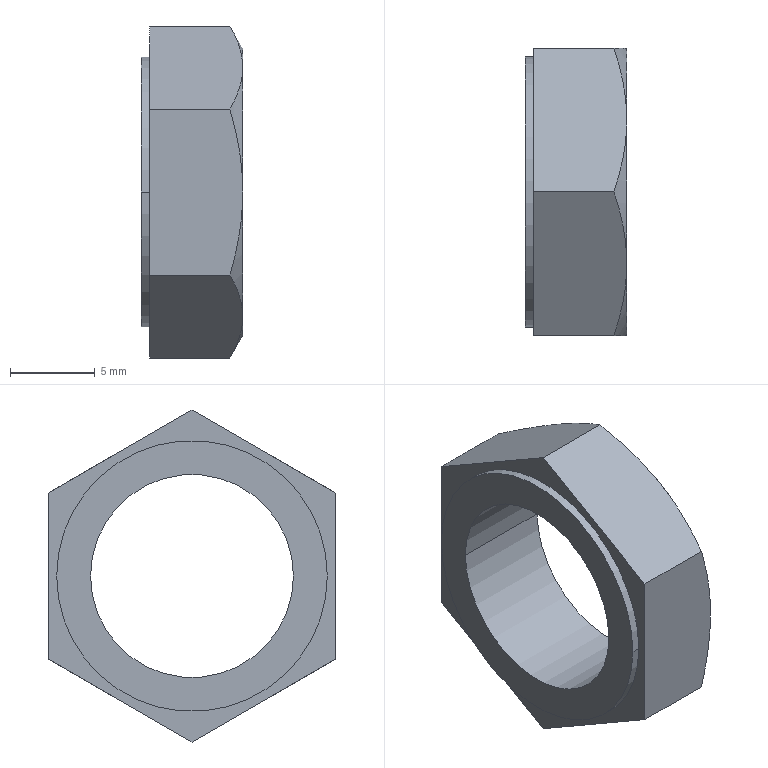Component | SolidWorks | MI10x10U(0)+()-1_MI10-M12x1_25 - Nut-1 | 1 solid | 19 faces | box 6 x 17 x 19.63 mm | volume 793 mm3 | plane 9 | cone 6 | cylinder 4 | commonest cylinder face diameters 12 x2 16 x2
build123d program:
from build123d import *

# Parameters (mm, degrees)
SKETCH2_W                         = 34
SKETCH2_H                         = 34
CUT_EXTRUDE1_DEPTH                = 12
SKETCH1_R                         = 6
M12_THREAD_MAJOR_DIA_RELIEF_DEPTH = 15.303


with BuildPart() as part:
    # Sketch1_2 → Revolve1 (revolve)
    with BuildSketch(Plane.XY, mode=Mode.PRIVATE) as revolve1_sk:
        Polygon((0, 0), (0, 8.5), (0.9815, 10.2), (5.5, 10.2), (5.5, 8), (6, 8), (6, 0), align=None)
    revolve(revolve1_sk.sketch.rotate(Axis((6, 0, 0), (-1, 0, 0)), 270), axis=Axis((6, 0, 0), (-1, 0, 0)))

    # Sketch2 → Cut-Extrude1 (cut)
    with BuildSketch(Plane(origin=(0, 0, 0), x_dir=(0, 0, -1), z_dir=(1, 0, 0))):
        Rectangle(SKETCH2_W, SKETCH2_H)
        Polygon((-8.5, -4.907), (0, -9.815), (8.5, -4.907), (8.5, 4.907), (0, 9.815), (-8.5, 4.907), align=None, mode=Mode.SUBTRACT)
    extrude(amount=CUT_EXTRUDE1_DEPTH, mode=Mode.SUBTRACT)

    # Sketch3 → Cut-Revolve1 (revolve, cut)
    with BuildSketch(Plane.XY, mode=Mode.PRIVATE) as cut_revolve1_sk:
        Polygon((0, 0), (0, 6), (0.6765, 5.324), (5.324, 5.324), (6, 6), (6, 0), align=None)
    revolve(cut_revolve1_sk.sketch.rotate(Axis((6, 0, 0), (-1, 0, 0)), 270), axis=Axis((6, 0, 0), (-1, 0, 0)), mode=Mode.SUBTRACT)

    # Sketch1 → M12 thread major-dia relief (cut, through all)
    with BuildSketch(Plane.ZY):
        Circle(SKETCH1_R)
    extrude(amount=-M12_THREAD_MAJOR_DIA_RELIEF_DEPTH, mode=Mode.SUBTRACT)


solid = part.part

# Placed as in the assembly
solid = solid.moved(Location((-7.325, 30.452, 72.77), (-90, 0, 180)))
STEP:
#1=CARTESIAN_POINT('',(-0.5246,0.9627,2.865));
#2=VERTEX_POINT('',#1);
#3=CARTESIAN_POINT('',(-0.5246,1.435,2.865));
#4=VERTEX_POINT('',#3);
#5=CARTESIAN_POINT('',(-0.5246,1.199,2.865));
#6=DIRECTION('',(1.,-0.,-0.));
#7=DIRECTION('',(0.,1.,0.));
#8=AXIS2_PLACEMENT_3D('',#5,#6,#7);
#9=CIRCLE('',#8,0.2362);
#10=EDGE_CURVE('',#2,#4,#9,.T.);
#11=ORIENTED_EDGE('',*,*,#10,.F.);
#12=CARTESIAN_POINT('',(-0.2884,0.9627,2.865));
#13=VERTEX_POINT('',#12);
#14=CARTESIAN_POINT('',(-0.5246,0.9627,2.865));
#15=DIRECTION('',(1.,-0.,-0.));
#16=VECTOR('',#15,39.37);
#17=LINE('',#14,#16);
#18=EDGE_CURVE('',#2,#13,#17,.T.);
#19=ORIENTED_EDGE('',*,*,#18,.T.);
#20=CARTESIAN_POINT('',(-0.2884,1.435,2.865));
#21=VERTEX_POINT('',#20);
#22=CARTESIAN_POINT('',(-0.2884,1.199,2.865));
#23=DIRECTION('',(1.,-0.,-0.));
#24=DIRECTION('',(0.,1.,0.));
#25=AXIS2_PLACEMENT_3D('',#22,#23,#24);
#26=CIRCLE('',#25,0.2362);
#27=EDGE_CURVE('',#13,#21,#26,.T.);
#28=ORIENTED_EDGE('',*,*,#27,.T.);
#29=CARTESIAN_POINT('',(-0.5246,1.435,2.865));
#30=DIRECTION('',(1.,-0.,-0.));
#31=VECTOR('',#30,39.37);
#32=LINE('',#29,#31);
#33=EDGE_CURVE('',#4,#21,#32,.T.);
#34=ORIENTED_EDGE('',*,*,#33,.F.);
#35=EDGE_LOOP('',(#11,#19,#28,#34));
#36=FACE_OUTER_BOUND('',#35,.T.);
#37=CARTESIAN_POINT('',(-0.5246,1.199,2.865));
#38=DIRECTION('',(1.,-0.,-0.));
#39=DIRECTION('',(0.,1.,0.));
#40=AXIS2_PLACEMENT_3D('',#37,#38,#39);
#41=CYLINDRICAL_SURFACE('',#40,0.2362);
#42=ADVANCED_FACE('',(#36),#41,.F.);
#43=CARTESIAN_POINT('',(-0.5246,1.514,2.865));
#44=VERTEX_POINT('',#43);
#45=CARTESIAN_POINT('',(-0.5246,0.8839,2.865));
#46=VERTEX_POINT('',#45);
#47=CARTESIAN_POINT('',(-0.5246,1.199,2.865));
#48=DIRECTION('',(1.,-0.,-0.));
#49=DIRECTION('',(0.,1.,0.));
#50=AXIS2_PLACEMENT_3D('',#47,#48,#49);
#51=CIRCLE('',#50,0.315);
#52=EDGE_CURVE('',#44,#46,#51,.T.);
#53=ORIENTED_EDGE('',*,*,#52,.T.);
#54=CARTESIAN_POINT('',(-0.5049,0.8839,2.865));
#55=VERTEX_POINT('',#54);
#56=CARTESIAN_POINT('',(-0.5246,0.8839,2.865));
#57=DIRECTION('',(1.,-0.,-0.));
#58=VECTOR('',#57,39.37);
#59=LINE('',#56,#58);
#60=EDGE_CURVE('',#46,#55,#59,.T.);
#61=ORIENTED_EDGE('',*,*,#60,.T.);
#62=CARTESIAN_POINT('',(-0.5049,1.514,2.865));
#63=VERTEX_POINT('',#62);
#64=CARTESIAN_POINT('',(-0.5049,1.199,2.865));
#65=DIRECTION('',(1.,-0.,-0.));
#66=DIRECTION('',(0.,1.,0.));
#67=AXIS2_PLACEMENT_3D('',#64,#65,#66);
#68=CIRCLE('',#67,0.315);
#69=EDGE_CURVE('',#63,#55,#68,.T.);
#70=ORIENTED_EDGE('',*,*,#69,.F.);
#71=CARTESIAN_POINT('',(-0.5246,1.514,2.865));
#72=DIRECTION('',(1.,-0.,-0.));
#73=VECTOR('',#72,39.37);
#74=LINE('',#71,#73);
#75=EDGE_CURVE('',#44,#63,#74,.T.);
#76=ORIENTED_EDGE('',*,*,#75,.F.);
#77=EDGE_LOOP('',(#53,#61,#70,#76));
#78=FACE_OUTER_BOUND('',#77,.T.);
#79=CARTESIAN_POINT('',(-0.5246,1.199,2.865));
#80=DIRECTION('',(1.,-0.,-0.));
#81=DIRECTION('',(0.,1.,0.));
#82=AXIS2_PLACEMENT_3D('',#79,#80,#81);
#83=CYLINDRICAL_SURFACE('',#82,0.315);
#84=ADVANCED_FACE('',(#78),#83,.T.);
#85=CARTESIAN_POINT('',(-0.5049,1.199,3.251));
#86=VERTEX_POINT('',#85);
#87=CARTESIAN_POINT('',(-0.5049,1.534,3.058));
#88=VERTEX_POINT('',#87);
#89=CARTESIAN_POINT('',(-0.5049,1.192,3.255));
#90=DIRECTION('',(0.,0.866,-0.5));
#91=VECTOR('',#90,39.37);
#92=LINE('',#89,#91);
#93=EDGE_CURVE('',#86,#88,#92,.T.);
#94=ORIENTED_EDGE('',*,*,#93,.T.);
#95=CARTESIAN_POINT('',(-0.5049,1.534,2.672));
#96=VERTEX_POINT('',#95);
#97=CARTESIAN_POINT('',(-0.5049,1.534,3.267));
#98=DIRECTION('',(-0.,0.,-1.));
#99=VECTOR('',#98,39.37);
#100=LINE('',#97,#99);
#101=EDGE_CURVE('',#88,#96,#100,.T.);
#102=ORIENTED_EDGE('',*,*,#101,.T.);
#103=CARTESIAN_POINT('',(-0.5049,1.199,2.479));
#104=VERTEX_POINT('',#103);
#105=CARTESIAN_POINT('',(-0.5049,1.54,2.676));
#106=DIRECTION('',(-0.,-0.866,-0.5));
#107=VECTOR('',#106,39.37);
#108=LINE('',#105,#107);
#109=EDGE_CURVE('',#96,#104,#108,.T.);
#110=ORIENTED_EDGE('',*,*,#109,.T.);
#111=CARTESIAN_POINT('',(-0.5049,0.8643,2.672));
#112=VERTEX_POINT('',#111);
#113=CARTESIAN_POINT('',(-0.5049,0.8577,2.676));
#114=DIRECTION('',(-0.,-0.866,0.5));
#115=VECTOR('',#114,39.37);
#116=LINE('',#113,#115);
#117=EDGE_CURVE('',#104,#112,#116,.T.);
#118=ORIENTED_EDGE('',*,*,#117,.T.);
#119=CARTESIAN_POINT('',(-0.5049,0.8643,3.058));
#120=VERTEX_POINT('',#119);
#121=CARTESIAN_POINT('',(-0.5049,0.8643,3.267));
#122=DIRECTION('',(0.,-0.,1.));
#123=VECTOR('',#122,39.37);
#124=LINE('',#121,#123);
#125=EDGE_CURVE('',#112,#120,#124,.T.);
#126=ORIENTED_EDGE('',*,*,#125,.T.);
#127=CARTESIAN_POINT('',(-0.5049,1.205,3.255));
#128=DIRECTION('',(0.,0.866,0.5));
#129=VECTOR('',#128,39.37);
#130=LINE('',#127,#129);
#131=EDGE_CURVE('',#120,#86,#130,.T.);
#132=ORIENTED_EDGE('',*,*,#131,.T.);
#133=EDGE_LOOP('',(#94,#102,#110,#118,#126,#132));
#134=FACE_OUTER_BOUND('',#133,.T.);
#135=ORIENTED_EDGE('',*,*,#69,.T.);
#136=CARTESIAN_POINT('',(-0.5049,1.199,2.865));
#137=DIRECTION('',(1.,-0.,-0.));
#138=DIRECTION('',(0.,1.,0.));
#139=AXIS2_PLACEMENT_3D('',#136,#137,#138);
#140=CIRCLE('',#139,0.315);
#141=EDGE_CURVE('',#55,#63,#140,.T.);
#142=ORIENTED_EDGE('',*,*,#141,.T.);
#143=EDGE_LOOP('',(#135,#142));
#144=FACE_BOUND('',#143,.T.);
#145=CARTESIAN_POINT('',(-0.5049,1.199,3.267));
#146=DIRECTION('',(1.,-0.,-0.));
#147=DIRECTION('',(0.,1.,0.));
#148=AXIS2_PLACEMENT_3D('',#145,#146,#147);
#149=PLANE('',#148);
#150=ADVANCED_FACE('',(#134,#144),#149,.F.);
#151=ORIENTED_EDGE('',*,*,#60,.F.);
#152=CARTESIAN_POINT('',(-0.5246,1.199,2.865));
#153=DIRECTION('',(1.,-0.,-0.));
#154=DIRECTION('',(0.,1.,0.));
#155=AXIS2_PLACEMENT_3D('',#152,#153,#154);
#156=CIRCLE('',#155,0.315);
#157=EDGE_CURVE('',#46,#44,#156,.T.);
#158=ORIENTED_EDGE('',*,*,#157,.T.);
#159=ORIENTED_EDGE('',*,*,#75,.T.);
#160=ORIENTED_EDGE('',*,*,#141,.F.);
#161=EDGE_LOOP('',(#151,#158,#159,#160));
#162=FACE_OUTER_BOUND('',#161,.T.);
#163=CARTESIAN_POINT('',(-0.5246,1.199,2.865));
#164=DIRECTION('',(1.,-0.,-0.));
#165=DIRECTION('',(0.,1.,0.));
#166=AXIS2_PLACEMENT_3D('',#163,#164,#165);
#167=CYLINDRICAL_SURFACE('',#166,0.315);
#168=ADVANCED_FACE('',(#162),#167,.T.);
#169=CARTESIAN_POINT('',(-0.5246,1.199,2.865));
#170=DIRECTION('',(1.,-0.,-0.));
#171=DIRECTION('',(0.,1.,0.));
#172=AXIS2_PLACEMENT_3D('',#169,#170,#171);
#173=CIRCLE('',#172,0.2362);
#174=EDGE_CURVE('',#4,#2,#173,.T.);
#175=ORIENTED_EDGE('',*,*,#174,.T.);
#176=ORIENTED_EDGE('',*,*,#10,.T.);
#177=EDGE_LOOP('',(#175,#176));
#178=FACE_BOUND('',#177,.T.);
#179=ORIENTED_EDGE('',*,*,#52,.F.);
#180=ORIENTED_EDGE('',*,*,#157,.F.);
#181=EDGE_LOOP('',(#179,#180));
#182=FACE_OUTER_BOUND('',#181,.T.);
#183=CARTESIAN_POINT('',(-0.5246,1.199,3.18));
#184=DIRECTION('',(1.,-0.,-0.));
#185=DIRECTION('',(0.,1.,0.));
#186=AXIS2_PLACEMENT_3D('',#183,#184,#185);
#187=PLANE('',#186);
#188=ADVANCED_FACE('',(#178,#182),#187,.F.);
#189=CARTESIAN_POINT('',(-0.3183,1.534,2.672));
#190=VERTEX_POINT('',#189);
#191=CARTESIAN_POINT('',(-0.7608,1.534,2.672));
#192=DIRECTION('',(1.,-0.,-0.));
#193=VECTOR('',#192,39.37);
#194=LINE('',#191,#193);
#195=EDGE_CURVE('',#96,#190,#194,.T.);
#196=ORIENTED_EDGE('',*,*,#195,.F.);
#197=ORIENTED_EDGE('',*,*,#101,.F.);
#198=CARTESIAN_POINT('',(-0.3183,1.534,3.058));
#199=VERTEX_POINT('',#198);
#200=CARTESIAN_POINT('',(-0.7608,1.534,3.058));
#201=DIRECTION('',(1.,-0.,-0.));
#202=VECTOR('',#201,39.37);
#203=LINE('',#200,#202);
#204=EDGE_CURVE('',#88,#199,#203,.T.);
#205=ORIENTED_EDGE('',*,*,#204,.T.);
#206=CARTESIAN_POINT('',(-0.2884,1.534,2.865));
#207=VERTEX_POINT('',#206);
#208=CARTESIAN_POINT('',(-0.2884,1.534,2.865));
#209=CARTESIAN_POINT('',(-0.2884,1.534,2.898));
#210=CARTESIAN_POINT('',(-0.2913,1.534,2.931));
#211=CARTESIAN_POINT('',(-0.3018,1.534,2.995));
#212=CARTESIAN_POINT('',(-0.3093,1.534,3.027));
#213=CARTESIAN_POINT('',(-0.3183,1.534,3.058));
#214=B_SPLINE_CURVE_WITH_KNOTS('',3,(#208,#209,#210,#211,#212,#213),.UNSPECIFIED.,.F.,.F.,(4,2,4),(0.01375,0.01624,0.01872),.UNSPECIFIED.);
#215=EDGE_CURVE('',#207,#199,#214,.T.);
#216=ORIENTED_EDGE('',*,*,#215,.F.);
#217=CARTESIAN_POINT('',(-0.3183,1.534,2.672));
#218=CARTESIAN_POINT('',(-0.3092,1.534,2.703));
#219=CARTESIAN_POINT('',(-0.3016,1.534,2.735));
#220=CARTESIAN_POINT('',(-0.2912,1.534,2.8));
#221=CARTESIAN_POINT('',(-0.2884,1.534,2.832));
#222=CARTESIAN_POINT('',(-0.2884,1.534,2.865));
#223=B_SPLINE_CURVE_WITH_KNOTS('',3,(#217,#218,#219,#220,#221,#222),.UNSPECIFIED.,.F.,.F.,(4,2,4),(0.00879,0.01127,0.01375),.UNSPECIFIED.);
#224=EDGE_CURVE('',#190,#207,#223,.T.);
#225=ORIENTED_EDGE('',*,*,#224,.F.);
#226=EDGE_LOOP('',(#196,#197,#205,#216,#225));
#227=FACE_OUTER_BOUND('',#226,.T.);
#228=CARTESIAN_POINT('',(-0.7608,1.534,3.058));
#229=DIRECTION('',(-0.,-1.,-0.));
#230=DIRECTION('',(1.,-0.,-0.));
#231=AXIS2_PLACEMENT_3D('',#228,#229,#230);
#232=PLANE('',#231);
#233=ADVANCED_FACE('',(#227),#232,.F.);
#234=CARTESIAN_POINT('',(-0.3183,1.199,2.479));
#235=VERTEX_POINT('',#234);
#236=CARTESIAN_POINT('',(-0.7608,1.199,2.479));
#237=DIRECTION('',(1.,-0.,-0.));
#238=VECTOR('',#237,39.37);
#239=LINE('',#236,#238);
#240=EDGE_CURVE('',#104,#235,#239,.T.);
#241=ORIENTED_EDGE('',*,*,#240,.F.);
#242=ORIENTED_EDGE('',*,*,#109,.F.);
#243=ORIENTED_EDGE('',*,*,#195,.T.);
#244=CARTESIAN_POINT('',(-0.2884,1.366,2.575));
#245=VERTEX_POINT('',#244);
#246=CARTESIAN_POINT('',(-0.2884,1.366,2.575));
#247=CARTESIAN_POINT('',(-0.2884,1.38,2.583));
#248=CARTESIAN_POINT('',(-0.2891,1.395,2.592));
#249=CARTESIAN_POINT('',(-0.2918,1.423,2.608));
#250=CARTESIAN_POINT('',(-0.2939,1.437,2.616));
#251=CARTESIAN_POINT('',(-0.3017,1.479,2.64));
#252=CARTESIAN_POINT('',(-0.3092,1.506,2.656));
#253=CARTESIAN_POINT('',(-0.3183,1.534,2.672));
#254=B_SPLINE_CURVE_WITH_KNOTS('',3,(#246,#247,#248,#249,#250,#251,#252,#253),.UNSPECIFIED.,.F.,.F.,(4,2,2,4),(0.004966,0.006203,0.007439,0.009913),.UNSPECIFIED.);
#255=EDGE_CURVE('',#245,#190,#254,.T.);
#256=ORIENTED_EDGE('',*,*,#255,.F.);
#257=CARTESIAN_POINT('',(-0.3183,1.199,2.479));
#258=CARTESIAN_POINT('',(-0.3092,1.226,2.494));
#259=CARTESIAN_POINT('',(-0.3017,1.254,2.51));
#260=CARTESIAN_POINT('',(-0.2913,1.31,2.542));
#261=CARTESIAN_POINT('',(-0.2884,1.338,2.559));
#262=CARTESIAN_POINT('',(-0.2884,1.366,2.575));
#263=B_SPLINE_CURVE_WITH_KNOTS('',3,(#257,#258,#259,#260,#261,#262),.UNSPECIFIED.,.F.,.F.,(4,2,4),(0.00000024,0.002483,0.004966),.UNSPECIFIED.);
#264=EDGE_CURVE('',#235,#245,#263,.T.);
#265=ORIENTED_EDGE('',*,*,#264,.F.);
#266=EDGE_LOOP('',(#241,#242,#243,#256,#265));
#267=FACE_OUTER_BOUND('',#266,.T.);
#268=CARTESIAN_POINT('',(-0.7608,1.534,2.672));
#269=DIRECTION('',(0.,-0.5,0.866));
#270=DIRECTION('',(0.,0.866,0.5));
#271=AXIS2_PLACEMENT_3D('',#268,#269,#270);
#272=PLANE('',#271);
#273=ADVANCED_FACE('',(#267),#272,.F.);
#274=CARTESIAN_POINT('',(-0.3183,0.8643,2.672));
#275=VERTEX_POINT('',#274);
#276=CARTESIAN_POINT('',(-0.7608,0.8643,2.672));
#277=DIRECTION('',(1.,-0.,-0.));
#278=VECTOR('',#277,39.37);
#279=LINE('',#276,#278);
#280=EDGE_CURVE('',#112,#275,#279,.T.);
#281=ORIENTED_EDGE('',*,*,#280,.F.);
#282=ORIENTED_EDGE('',*,*,#117,.F.);
#283=ORIENTED_EDGE('',*,*,#240,.T.);
#284=CARTESIAN_POINT('',(-0.2884,1.032,2.575));
#285=VERTEX_POINT('',#284);
#286=CARTESIAN_POINT('',(-0.2884,1.032,2.575));
#287=CARTESIAN_POINT('',(-0.2884,1.046,2.567));
#288=CARTESIAN_POINT('',(-0.2891,1.06,2.559));
#289=CARTESIAN_POINT('',(-0.2918,1.088,2.542));
#290=CARTESIAN_POINT('',(-0.2939,1.102,2.534));
#291=CARTESIAN_POINT('',(-0.3017,1.144,2.51));
#292=CARTESIAN_POINT('',(-0.3092,1.172,2.494));
#293=CARTESIAN_POINT('',(-0.3183,1.199,2.479));
#294=B_SPLINE_CURVE_WITH_KNOTS('',3,(#286,#287,#288,#289,#290,#291,#292,#293),.UNSPECIFIED.,.F.,.F.,(4,2,2,4),(0.004966,0.006203,0.007439,0.009913),.UNSPECIFIED.);
#295=EDGE_CURVE('',#285,#235,#294,.T.);
#296=ORIENTED_EDGE('',*,*,#295,.F.);
#297=CARTESIAN_POINT('',(-0.3183,0.8643,2.672));
#298=CARTESIAN_POINT('',(-0.3092,0.8916,2.656));
#299=CARTESIAN_POINT('',(-0.3017,0.9192,2.64));
#300=CARTESIAN_POINT('',(-0.2913,0.9749,2.608));
#301=CARTESIAN_POINT('',(-0.2884,1.003,2.592));
#302=CARTESIAN_POINT('',(-0.2884,1.032,2.575));
#303=B_SPLINE_CURVE_WITH_KNOTS('',3,(#297,#298,#299,#300,#301,#302),.UNSPECIFIED.,.F.,.F.,(4,2,4),(0.00000024,0.002483,0.004966),.UNSPECIFIED.);
#304=EDGE_CURVE('',#275,#285,#303,.T.);
#305=ORIENTED_EDGE('',*,*,#304,.F.);
#306=EDGE_LOOP('',(#281,#282,#283,#296,#305));
#307=FACE_OUTER_BOUND('',#306,.T.);
#308=CARTESIAN_POINT('',(-0.7608,1.199,2.479));
#309=DIRECTION('',(0.,0.5,0.866));
#310=DIRECTION('',(0.,0.866,-0.5));
#311=AXIS2_PLACEMENT_3D('',#308,#309,#310);
#312=PLANE('',#311);
#313=ADVANCED_FACE('',(#307),#312,.F.);
#314=CARTESIAN_POINT('',(-0.3183,0.8643,3.058));
#315=VERTEX_POINT('',#314);
#316=CARTESIAN_POINT('',(-0.7608,0.8643,3.058));
#317=DIRECTION('',(1.,-0.,-0.));
#318=VECTOR('',#317,39.37);
#319=LINE('',#316,#318);
#320=EDGE_CURVE('',#120,#315,#319,.T.);
#321=ORIENTED_EDGE('',*,*,#320,.F.);
#322=ORIENTED_EDGE('',*,*,#125,.F.);
#323=ORIENTED_EDGE('',*,*,#280,.T.);
#324=CARTESIAN_POINT('',(-0.2884,0.8643,2.865));
#325=VERTEX_POINT('',#324);
#326=CARTESIAN_POINT('',(-0.2884,0.8643,2.865));
#327=CARTESIAN_POINT('',(-0.2884,0.8643,2.832));
#328=CARTESIAN_POINT('',(-0.2912,0.8643,2.8));
#329=CARTESIAN_POINT('',(-0.3016,0.8643,2.735));
#330=CARTESIAN_POINT('',(-0.3092,0.8643,2.703));
#331=CARTESIAN_POINT('',(-0.3183,0.8643,2.672));
#332=B_SPLINE_CURVE_WITH_KNOTS('',3,(#326,#327,#328,#329,#330,#331),.UNSPECIFIED.,.F.,.F.,(4,2,4),(0.02652,0.029,0.03149),.UNSPECIFIED.);
#333=EDGE_CURVE('',#325,#275,#332,.T.);
#334=ORIENTED_EDGE('',*,*,#333,.F.);
#335=CARTESIAN_POINT('',(-0.3183,0.8643,3.058));
#336=CARTESIAN_POINT('',(-0.3093,0.8643,3.027));
#337=CARTESIAN_POINT('',(-0.3018,0.8643,2.995));
#338=CARTESIAN_POINT('',(-0.2913,0.8643,2.931));
#339=CARTESIAN_POINT('',(-0.2884,0.8643,2.898));
#340=CARTESIAN_POINT('',(-0.2884,0.8643,2.865));
#341=B_SPLINE_CURVE_WITH_KNOTS('',3,(#335,#336,#337,#338,#339,#340),.UNSPECIFIED.,.F.,.F.,(4,2,4),(0.02154,0.02403,0.02652),.UNSPECIFIED.);
#342=EDGE_CURVE('',#315,#325,#341,.T.);
#343=ORIENTED_EDGE('',*,*,#342,.F.);
#344=EDGE_LOOP('',(#321,#322,#323,#334,#343));
#345=FACE_OUTER_BOUND('',#344,.T.);
#346=CARTESIAN_POINT('',(-0.7608,0.8643,2.672));
#347=DIRECTION('',(0.,1.,0.));
#348=DIRECTION('',(-1.,0.,0.));
#349=AXIS2_PLACEMENT_3D('',#346,#347,#348);
#350=PLANE('',#349);
#351=ADVANCED_FACE('',(#345),#350,.F.);
#352=CARTESIAN_POINT('',(-0.3183,1.199,3.251));
#353=VERTEX_POINT('',#352);
#354=CARTESIAN_POINT('',(-0.7608,1.199,3.251));
#355=DIRECTION('',(1.,-0.,-0.));
#356=VECTOR('',#355,39.37);
#357=LINE('',#354,#356);
#358=EDGE_CURVE('',#86,#353,#357,.T.);
#359=ORIENTED_EDGE('',*,*,#358,.F.);
#360=ORIENTED_EDGE('',*,*,#131,.F.);
#361=ORIENTED_EDGE('',*,*,#320,.T.);
#362=CARTESIAN_POINT('',(-0.2884,1.032,3.155));
#363=VERTEX_POINT('',#362);
#364=CARTESIAN_POINT('',(-0.2884,1.032,3.155));
#365=CARTESIAN_POINT('',(-0.2884,1.017,3.147));
#366=CARTESIAN_POINT('',(-0.2891,1.003,3.138));
#367=CARTESIAN_POINT('',(-0.2918,0.9749,3.122));
#368=CARTESIAN_POINT('',(-0.2939,0.9609,3.114));
#369=CARTESIAN_POINT('',(-0.3017,0.9191,3.09));
#370=CARTESIAN_POINT('',(-0.3092,0.8916,3.074));
#371=CARTESIAN_POINT('',(-0.3183,0.8643,3.058));
#372=B_SPLINE_CURVE_WITH_KNOTS('',3,(#364,#365,#366,#367,#368,#369,#370,#371),.UNSPECIFIED.,.F.,.F.,(4,2,2,4),(0.004966,0.006203,0.007439,0.009913),.UNSPECIFIED.);
#373=EDGE_CURVE('',#363,#315,#372,.T.);
#374=ORIENTED_EDGE('',*,*,#373,.F.);
#375=CARTESIAN_POINT('',(-0.3183,1.199,3.251));
#376=CARTESIAN_POINT('',(-0.3092,1.172,3.236));
#377=CARTESIAN_POINT('',(-0.3017,1.144,3.22));
#378=CARTESIAN_POINT('',(-0.2913,1.088,3.187));
#379=CARTESIAN_POINT('',(-0.2884,1.06,3.171));
#380=CARTESIAN_POINT('',(-0.2884,1.032,3.155));
#381=B_SPLINE_CURVE_WITH_KNOTS('',3,(#375,#376,#377,#378,#379,#380),.UNSPECIFIED.,.F.,.F.,(4,2,4),(0.00000024,0.002483,0.004966),.UNSPECIFIED.);
#382=EDGE_CURVE('',#353,#363,#381,.T.);
#383=ORIENTED_EDGE('',*,*,#382,.F.);
#384=EDGE_LOOP('',(#359,#360,#361,#374,#383));
#385=FACE_OUTER_BOUND('',#384,.T.);
#386=CARTESIAN_POINT('',(-0.7608,0.8643,3.058));
#387=DIRECTION('',(-0.,0.5,-0.866));
#388=DIRECTION('',(-0.,-0.866,-0.5));
#389=AXIS2_PLACEMENT_3D('',#386,#387,#388);
#390=PLANE('',#389);
#391=ADVANCED_FACE('',(#385),#390,.F.);
#392=ORIENTED_EDGE('',*,*,#204,.F.);
#393=ORIENTED_EDGE('',*,*,#93,.F.);
#394=ORIENTED_EDGE('',*,*,#358,.T.);
#395=CARTESIAN_POINT('',(-0.2884,1.366,3.155));
#396=VERTEX_POINT('',#395);
#397=CARTESIAN_POINT('',(-0.2884,1.366,3.155));
#398=CARTESIAN_POINT('',(-0.2884,1.352,3.163));
#399=CARTESIAN_POINT('',(-0.2891,1.338,3.171));
#400=CARTESIAN_POINT('',(-0.2918,1.31,3.187));
#401=CARTESIAN_POINT('',(-0.2939,1.296,3.196));
#402=CARTESIAN_POINT('',(-0.3017,1.254,3.22));
#403=CARTESIAN_POINT('',(-0.3092,1.226,3.236));
#404=CARTESIAN_POINT('',(-0.3183,1.199,3.251));
#405=B_SPLINE_CURVE_WITH_KNOTS('',3,(#397,#398,#399,#400,#401,#402,#403,#404),.UNSPECIFIED.,.F.,.F.,(4,2,2,4),(0.004966,0.006203,0.007439,0.009913),.UNSPECIFIED.);
#406=EDGE_CURVE('',#396,#353,#405,.T.);
#407=ORIENTED_EDGE('',*,*,#406,.F.);
#408=CARTESIAN_POINT('',(-0.3183,1.534,3.058));
#409=CARTESIAN_POINT('',(-0.3092,1.506,3.074));
#410=CARTESIAN_POINT('',(-0.3017,1.479,3.09));
#411=CARTESIAN_POINT('',(-0.2913,1.423,3.122));
#412=CARTESIAN_POINT('',(-0.2884,1.395,3.138));
#413=CARTESIAN_POINT('',(-0.2884,1.366,3.155));
#414=B_SPLINE_CURVE_WITH_KNOTS('',3,(#408,#409,#410,#411,#412,#413),.UNSPECIFIED.,.F.,.F.,(4,2,4),(0.00000024,0.002483,0.004966),.UNSPECIFIED.);
#415=EDGE_CURVE('',#199,#396,#414,.T.);
#416=ORIENTED_EDGE('',*,*,#415,.F.);
#417=EDGE_LOOP('',(#392,#393,#394,#407,#416));
#418=FACE_OUTER_BOUND('',#417,.T.);
#419=CARTESIAN_POINT('',(-0.7608,1.199,3.251));
#420=DIRECTION('',(-0.,-0.5,-0.866));
#421=DIRECTION('',(-0.,-0.866,0.5));
#422=AXIS2_PLACEMENT_3D('',#419,#420,#421);
#423=PLANE('',#422);
#424=ADVANCED_FACE('',(#418),#423,.F.);
#425=CARTESIAN_POINT('',(-0.2884,1.199,2.865));
#426=DIRECTION('',(1.,-0.,-0.));
#427=DIRECTION('',(0.,1.,0.));
#428=AXIS2_PLACEMENT_3D('',#425,#426,#427);
#429=CIRCLE('',#428,0.3346);
#430=EDGE_CURVE('',#245,#207,#429,.T.);
#431=ORIENTED_EDGE('',*,*,#430,.F.);
#432=ORIENTED_EDGE('',*,*,#255,.T.);
#433=ORIENTED_EDGE('',*,*,#224,.T.);
#434=EDGE_LOOP('',(#431,#432,#433));
#435=FACE_OUTER_BOUND('',#434,.T.);
#436=CARTESIAN_POINT('',(-0.327,1.199,2.865));
#437=DIRECTION('',(-1.,0.,0.));
#438=DIRECTION('',(-0.,-1.,0.));
#439=AXIS2_PLACEMENT_3D('',#436,#437,#438);
#440=CONICAL_SURFACE('',#439,0.4016,1.047);
#441=ADVANCED_FACE('',(#435),#440,.T.);
#442=CARTESIAN_POINT('',(-0.2884,1.199,2.865));
#443=DIRECTION('',(1.,-0.,-0.));
#444=DIRECTION('',(0.,1.,0.));
#445=AXIS2_PLACEMENT_3D('',#442,#443,#444);
#446=CIRCLE('',#445,0.3346);
#447=EDGE_CURVE('',#285,#245,#446,.T.);
#448=ORIENTED_EDGE('',*,*,#447,.F.);
#449=ORIENTED_EDGE('',*,*,#295,.T.);
#450=ORIENTED_EDGE('',*,*,#264,.T.);
#451=EDGE_LOOP('',(#448,#449,#450));
#452=FACE_OUTER_BOUND('',#451,.T.);
#453=CARTESIAN_POINT('',(-0.327,1.199,2.865));
#454=DIRECTION('',(-1.,0.,0.));
#455=DIRECTION('',(-0.,-1.,0.));
#456=AXIS2_PLACEMENT_3D('',#453,#454,#455);
#457=CONICAL_SURFACE('',#456,0.4016,1.047);
#458=ADVANCED_FACE('',(#452),#457,.T.);
#459=ORIENTED_EDGE('',*,*,#333,.T.);
#460=ORIENTED_EDGE('',*,*,#304,.T.);
#461=CARTESIAN_POINT('',(-0.2884,1.199,2.865));
#462=DIRECTION('',(1.,-0.,-0.));
#463=DIRECTION('',(0.,1.,0.));
#464=AXIS2_PLACEMENT_3D('',#461,#462,#463);
#465=CIRCLE('',#464,0.3346);
#466=EDGE_CURVE('',#325,#285,#465,.T.);
#467=ORIENTED_EDGE('',*,*,#466,.F.);
#468=EDGE_LOOP('',(#459,#460,#467));
#469=FACE_OUTER_BOUND('',#468,.T.);
#470=CARTESIAN_POINT('',(-0.327,1.199,2.865));
#471=DIRECTION('',(-1.,0.,0.));
#472=DIRECTION('',(-0.,-1.,0.));
#473=AXIS2_PLACEMENT_3D('',#470,#471,#472);
#474=CONICAL_SURFACE('',#473,0.4016,1.047);
#475=ADVANCED_FACE('',(#469),#474,.T.);
#476=ORIENTED_EDGE('',*,*,#373,.T.);
#477=ORIENTED_EDGE('',*,*,#342,.T.);
#478=CARTESIAN_POINT('',(-0.2884,1.199,2.865));
#479=DIRECTION('',(1.,-0.,-0.));
#480=DIRECTION('',(0.,1.,0.));
#481=AXIS2_PLACEMENT_3D('',#478,#479,#480);
#482=CIRCLE('',#481,0.3346);
#483=EDGE_CURVE('',#363,#325,#482,.T.);
#484=ORIENTED_EDGE('',*,*,#483,.F.);
#485=EDGE_LOOP('',(#476,#477,#484));
#486=FACE_OUTER_BOUND('',#485,.T.);
#487=CARTESIAN_POINT('',(-0.327,1.199,2.865));
#488=DIRECTION('',(-1.,0.,0.));
#489=DIRECTION('',(-0.,-1.,0.));
#490=AXIS2_PLACEMENT_3D('',#487,#488,#489);
#491=CONICAL_SURFACE('',#490,0.4016,1.047);
#492=ADVANCED_FACE('',(#486),#491,.T.);
#493=CARTESIAN_POINT('',(-0.2884,1.199,2.865));
#494=DIRECTION('',(1.,-0.,-0.));
#495=DIRECTION('',(0.,1.,0.));
#496=AXIS2_PLACEMENT_3D('',#493,#494,#495);
#497=CIRCLE('',#496,0.3346);
#498=EDGE_CURVE('',#207,#396,#497,.T.);
#499=ORIENTED_EDGE('',*,*,#498,.F.);
#500=ORIENTED_EDGE('',*,*,#215,.T.);
#501=ORIENTED_EDGE('',*,*,#415,.T.);
#502=EDGE_LOOP('',(#499,#500,#501));
#503=FACE_OUTER_BOUND('',#502,.T.);
#504=CARTESIAN_POINT('',(-0.327,1.199,2.865));
#505=DIRECTION('',(-1.,0.,0.));
#506=DIRECTION('',(-0.,-1.,0.));
#507=AXIS2_PLACEMENT_3D('',#504,#505,#506);
#508=CONICAL_SURFACE('',#507,0.4016,1.047);
#509=ADVANCED_FACE('',(#503),#508,.T.);
#510=CARTESIAN_POINT('',(-0.2884,1.199,2.865));
#511=DIRECTION('',(1.,-0.,-0.));
#512=DIRECTION('',(0.,1.,0.));
#513=AXIS2_PLACEMENT_3D('',#510,#511,#512);
#514=CIRCLE('',#513,0.2362);
#515=EDGE_CURVE('',#21,#13,#514,.T.);
#516=ORIENTED_EDGE('',*,*,#515,.F.);
#517=ORIENTED_EDGE('',*,*,#27,.F.);
#518=EDGE_LOOP('',(#516,#517));
#519=FACE_BOUND('',#518,.T.);
#520=ORIENTED_EDGE('',*,*,#498,.T.);
#521=CARTESIAN_POINT('',(-0.2884,1.199,2.865));
#522=DIRECTION('',(1.,-0.,-0.));
#523=DIRECTION('',(0.,1.,0.));
#524=AXIS2_PLACEMENT_3D('',#521,#522,#523);
#525=CIRCLE('',#524,0.3346);
#526=EDGE_CURVE('',#396,#363,#525,.T.);
#527=ORIENTED_EDGE('',*,*,#526,.T.);
#528=ORIENTED_EDGE('',*,*,#483,.T.);
#529=ORIENTED_EDGE('',*,*,#466,.T.);
#530=ORIENTED_EDGE('',*,*,#447,.T.);
#531=ORIENTED_EDGE('',*,*,#430,.T.);
#532=EDGE_LOOP('',(#520,#527,#528,#529,#530,#531));
#533=FACE_OUTER_BOUND('',#532,.T.);
#534=CARTESIAN_POINT('',(-0.2884,1.199,2.865));
#535=DIRECTION('',(-1.,0.,0.));
#536=DIRECTION('',(-0.,-1.,-0.));
#537=AXIS2_PLACEMENT_3D('',#534,#535,#536);
#538=PLANE('',#537);
#539=ADVANCED_FACE('',(#519,#533),#538,.F.);
#540=ORIENTED_EDGE('',*,*,#406,.T.);
#541=ORIENTED_EDGE('',*,*,#382,.T.);
#542=ORIENTED_EDGE('',*,*,#526,.F.);
#543=EDGE_LOOP('',(#540,#541,#542));
#544=FACE_OUTER_BOUND('',#543,.T.);
#545=CARTESIAN_POINT('',(-0.327,1.199,2.865));
#546=DIRECTION('',(-1.,0.,0.));
#547=DIRECTION('',(-0.,-1.,0.));
#548=AXIS2_PLACEMENT_3D('',#545,#546,#547);
#549=CONICAL_SURFACE('',#548,0.4016,1.047);
#550=ADVANCED_FACE('',(#544),#549,.T.);
#551=ORIENTED_EDGE('',*,*,#18,.F.);
#552=ORIENTED_EDGE('',*,*,#174,.F.);
#553=ORIENTED_EDGE('',*,*,#33,.T.);
#554=ORIENTED_EDGE('',*,*,#515,.T.);
#555=EDGE_LOOP('',(#551,#552,#553,#554));
#556=FACE_OUTER_BOUND('',#555,.T.);
#557=CARTESIAN_POINT('',(-0.5246,1.199,2.865));
#558=DIRECTION('',(1.,-0.,-0.));
#559=DIRECTION('',(0.,1.,0.));
#560=AXIS2_PLACEMENT_3D('',#557,#558,#559);
#561=CYLINDRICAL_SURFACE('',#560,0.2362);
#562=ADVANCED_FACE('',(#556),#561,.F.);
#563=CLOSED_SHELL('',(#42,#84,#150,#168,#188,#233,#273,#313,#351,#391,#424,#441,#458,#475,#492,#509,#539,#550,#562));
#564=MANIFOLD_SOLID_BREP('',#563);
#565=CARTESIAN_POINT('',(0.,0.,0.));
#566=DIRECTION('',(0.,0.,1.));
#567=DIRECTION('',(1.,0.,0.));
#568=AXIS2_PLACEMENT_3D('',#565,#566,#567);
#569=(LENGTH_UNIT()NAMED_UNIT(*)SI_UNIT($,.METRE.));
#570=LENGTH_MEASURE_WITH_UNIT(LENGTH_MEASURE(0.0254),#569);
#571=DIMENSIONAL_EXPONENTS(1.,0.,0.,0.,0.,0.,0.);
#572=(CONVERSION_BASED_UNIT('',#570)LENGTH_UNIT()NAMED_UNIT(#571));
#573=UNCERTAINTY_MEASURE_WITH_UNIT(LENGTH_MEASURE(0.00001),#572,'','');
#574=(NAMED_UNIT(*)PLANE_ANGLE_UNIT()SI_UNIT($,.RADIAN.));
#575=(NAMED_UNIT(*)SI_UNIT($,.STERADIAN.)SOLID_ANGLE_UNIT());
#576=(GEOMETRIC_REPRESENTATION_CONTEXT(3)GLOBAL_UNCERTAINTY_ASSIGNED_CONTEXT((#573))GLOBAL_UNIT_ASSIGNED_CONTEXT((#572,#574,#575))REPRESENTATION_CONTEXT('',''));
#577=ADVANCED_BREP_SHAPE_REPRESENTATION('',(#564,#568),#576);
#578=COLOUR_RGB('',0.7922,0.8196,0.9333);
#579=FILL_AREA_STYLE_COLOUR('',#578);
#580=FILL_AREA_STYLE('',(#579));
#581=SURFACE_STYLE_FILL_AREA(#580);
#582=SURFACE_SIDE_STYLE('',(#581));
#583=SURFACE_STYLE_USAGE(.BOTH.,#582);
#584=PRESENTATION_STYLE_ASSIGNMENT((#583));
#585=STYLED_ITEM('',(#584),#564);
#586=PRESENTATION_LAYER_ASSIGNMENT('','',(#585));
#587=(LENGTH_UNIT()NAMED_UNIT(*)SI_UNIT($,.METRE.));
#588=LENGTH_MEASURE_WITH_UNIT(LENGTH_MEASURE(0.0254),#587);
#589=DIMENSIONAL_EXPONENTS(1.,0.,0.,0.,0.,0.,0.);
#590=(CONVERSION_BASED_UNIT('',#588)LENGTH_UNIT()NAMED_UNIT(#589));
#591=UNCERTAINTY_MEASURE_WITH_UNIT(LENGTH_MEASURE(0.00001),#590,'','');
#592=(NAMED_UNIT(*)PLANE_ANGLE_UNIT()SI_UNIT($,.RADIAN.));
#593=(NAMED_UNIT(*)SI_UNIT($,.STERADIAN.)SOLID_ANGLE_UNIT());
#594=(GEOMETRIC_REPRESENTATION_CONTEXT(3)GLOBAL_UNCERTAINTY_ASSIGNED_CONTEXT((#591))GLOBAL_UNIT_ASSIGNED_CONTEXT((#590,#592,#593))REPRESENTATION_CONTEXT('',''));
#595=MECHANICAL_DESIGN_GEOMETRIC_PRESENTATION_REPRESENTATION('',(#585),#594);